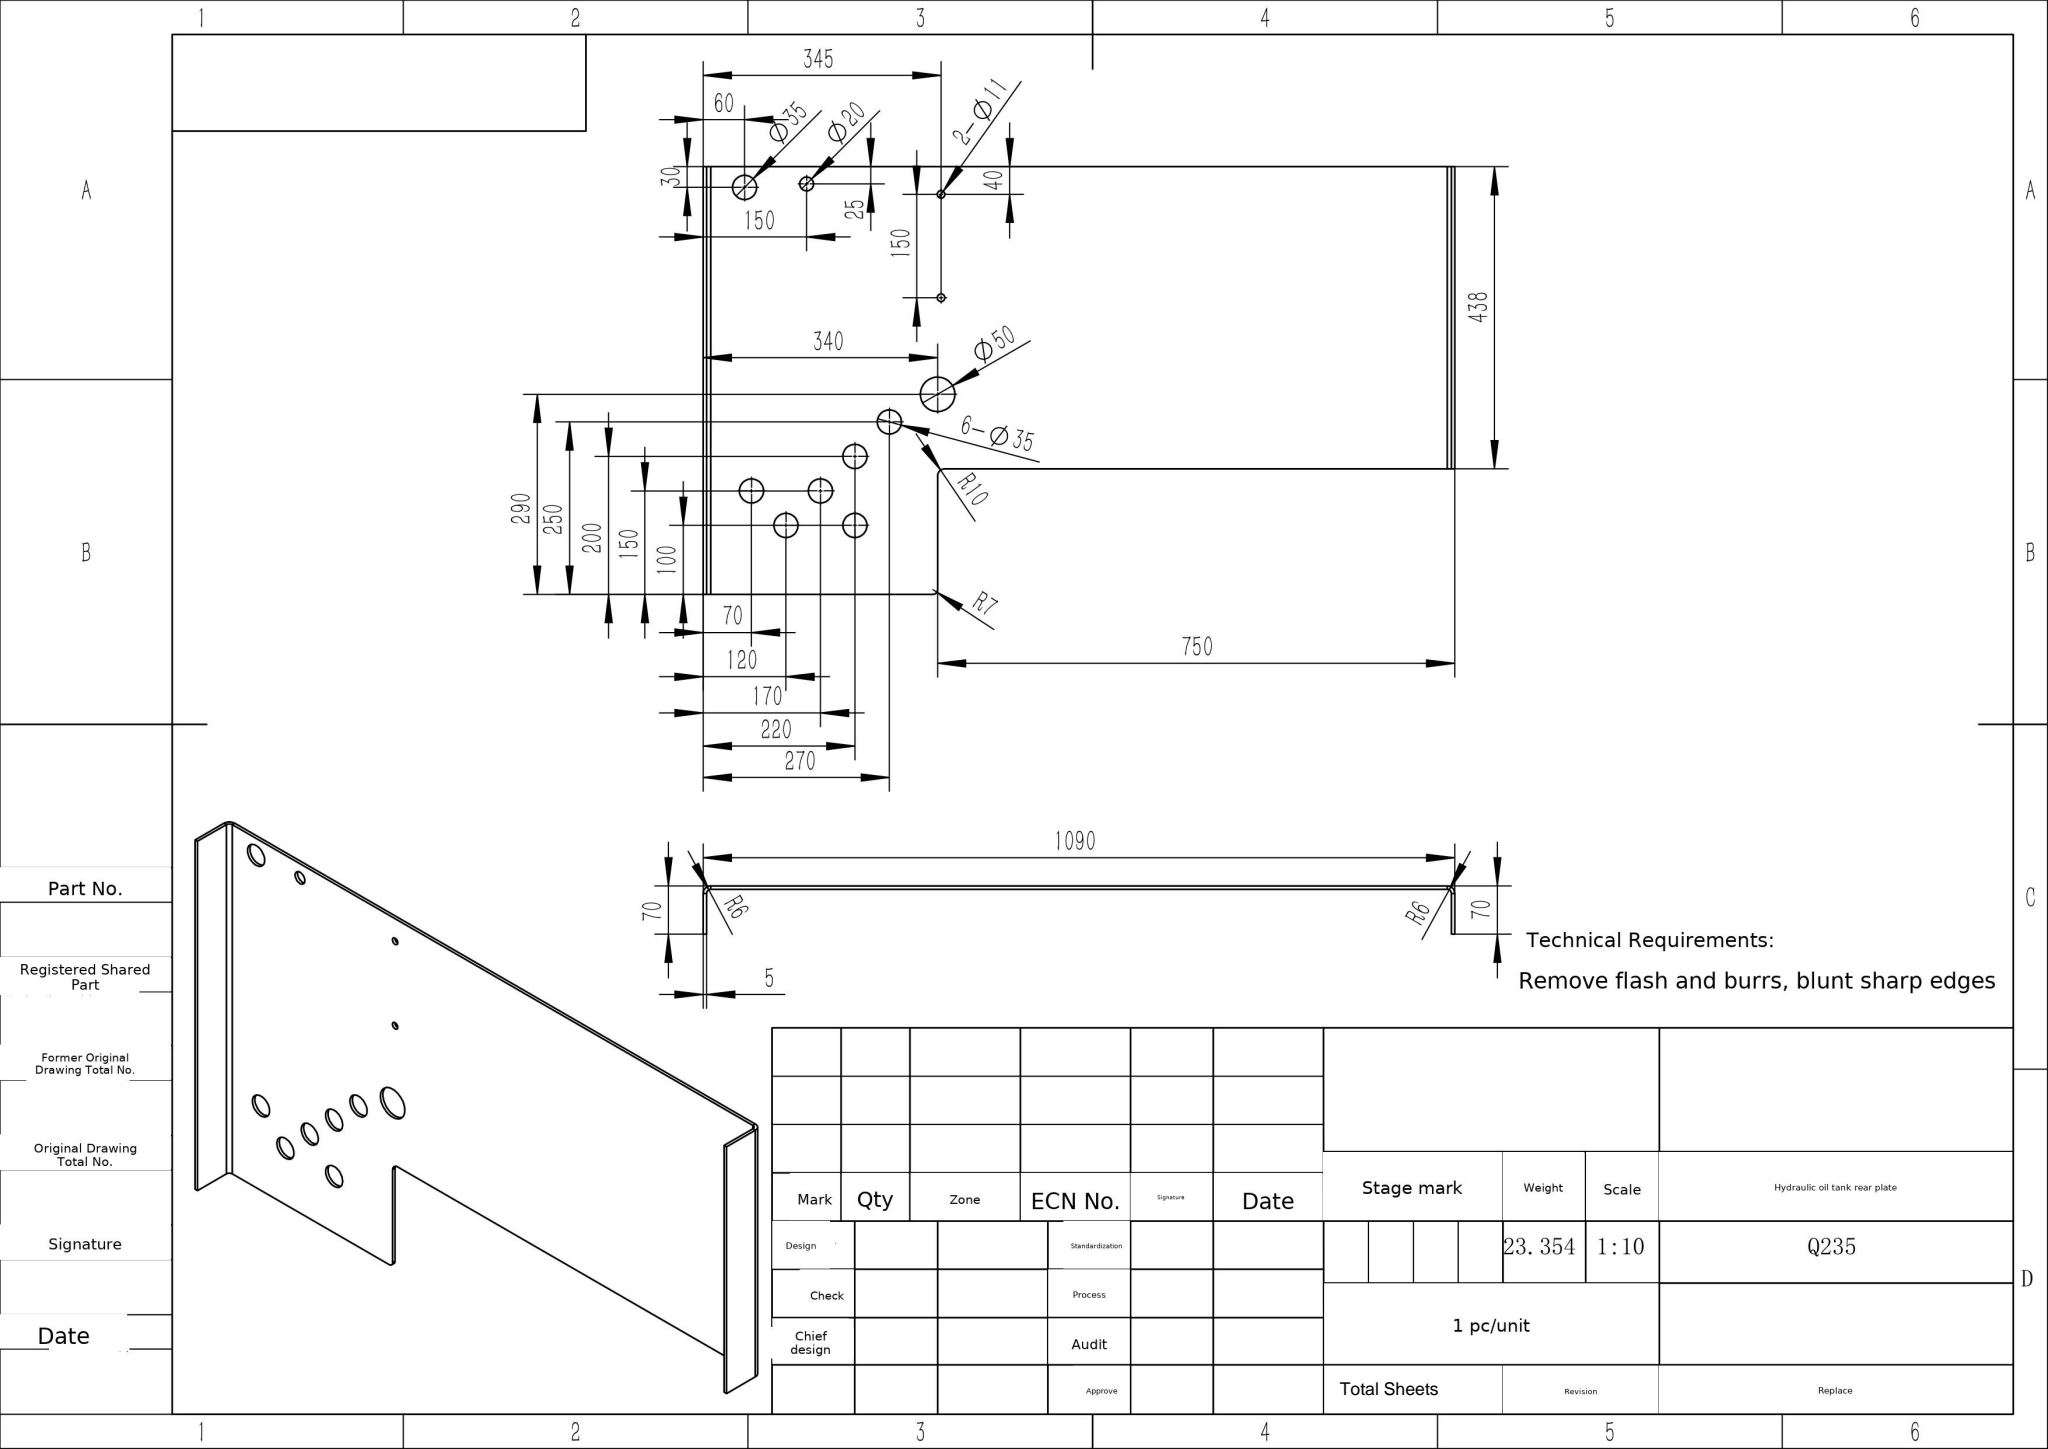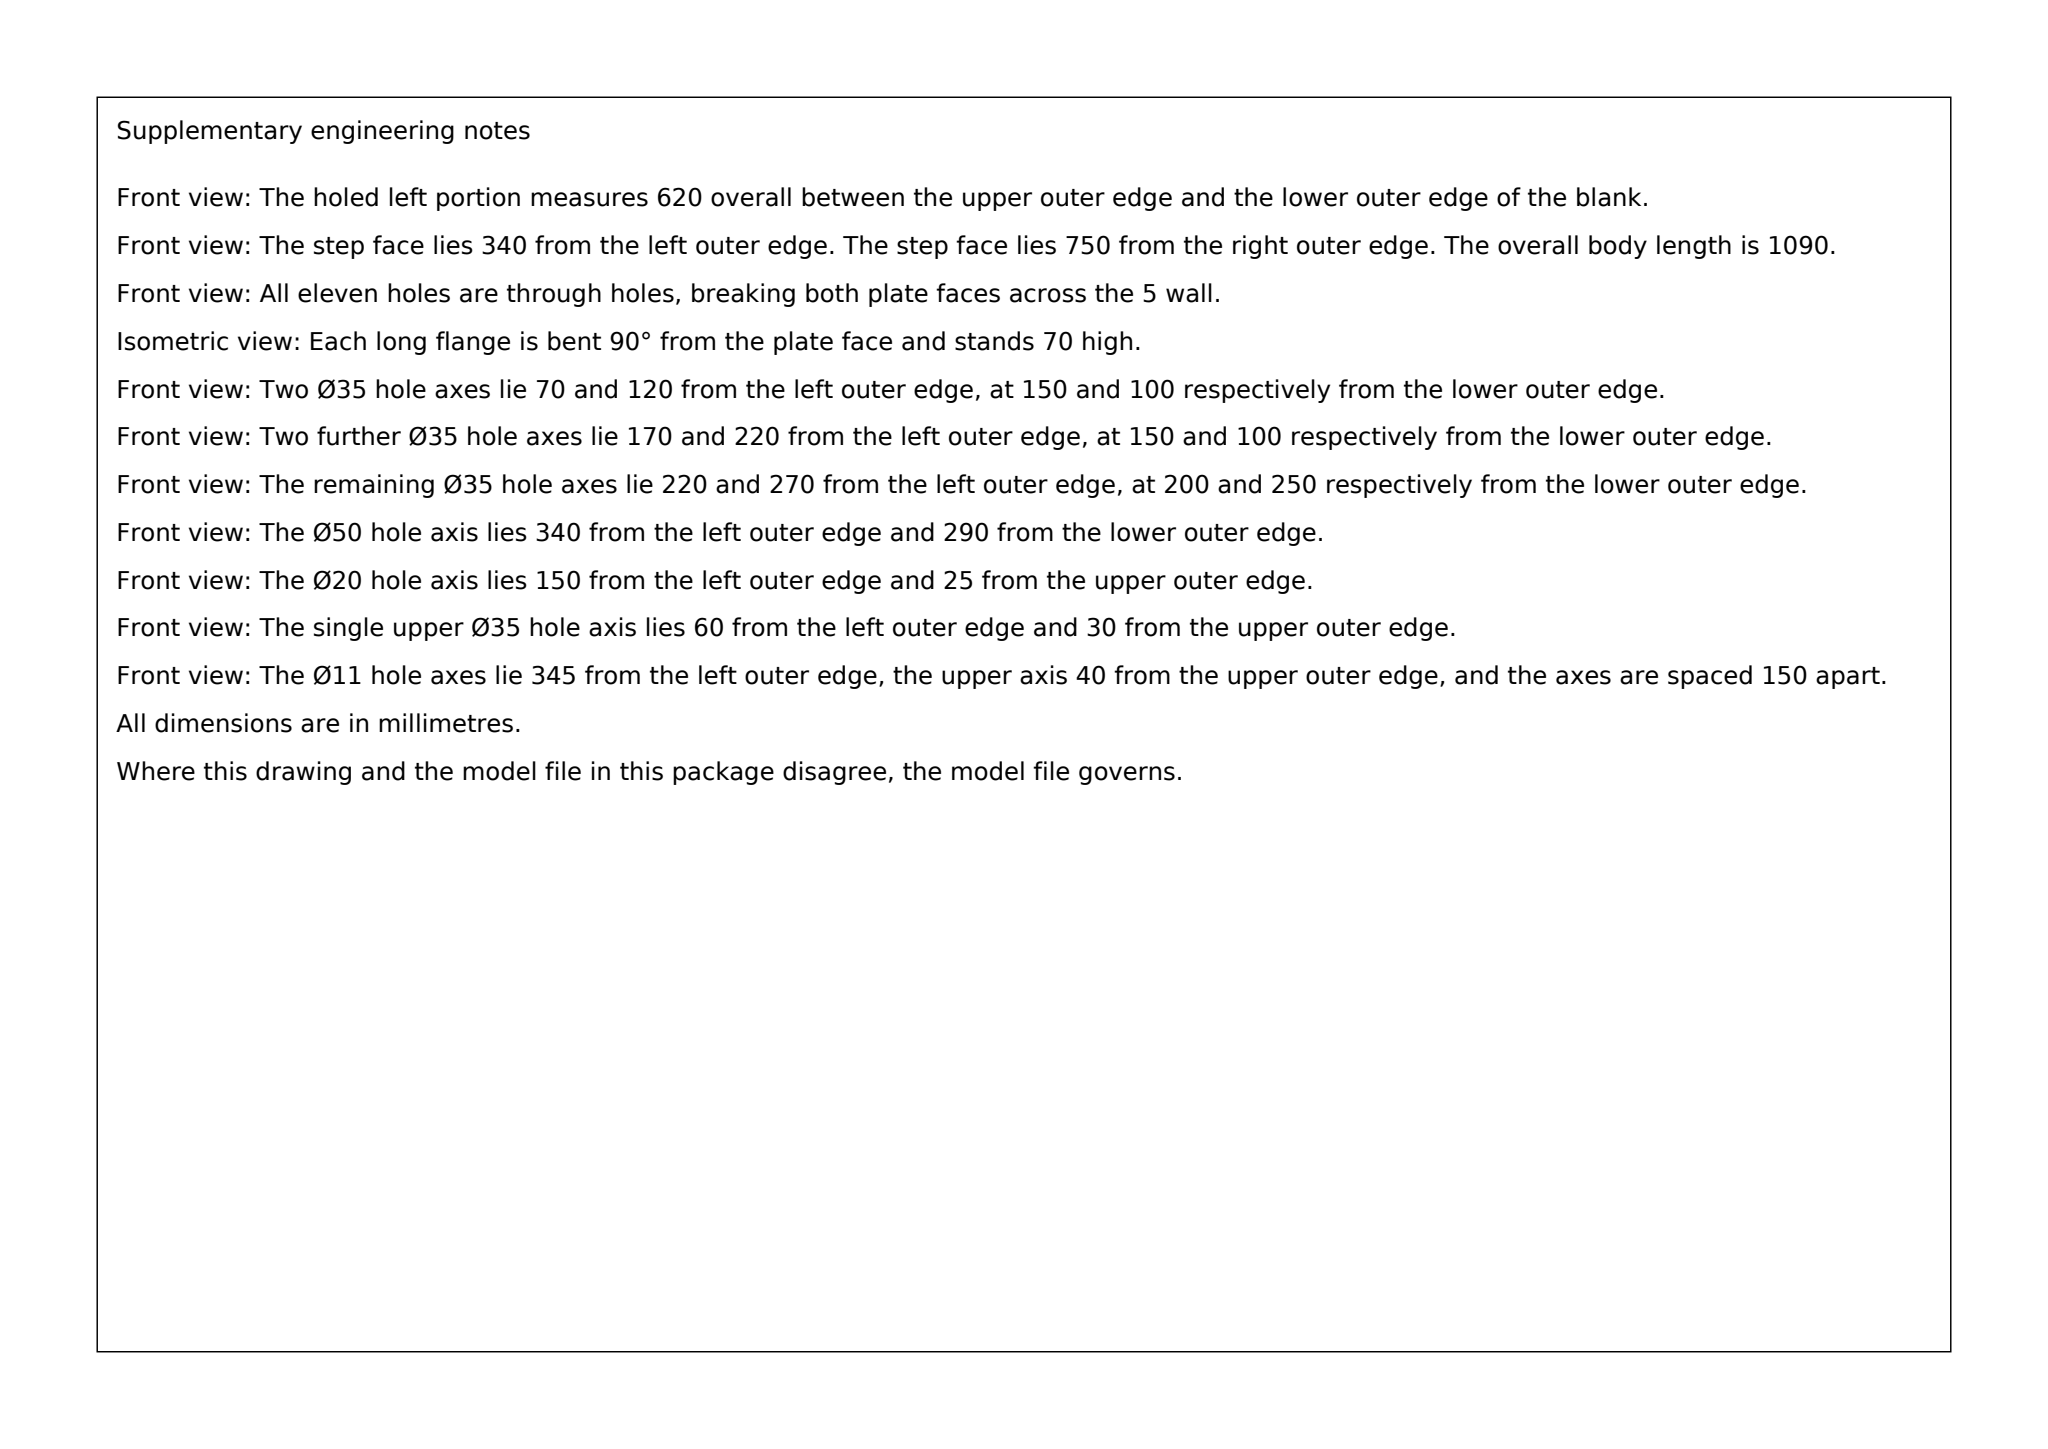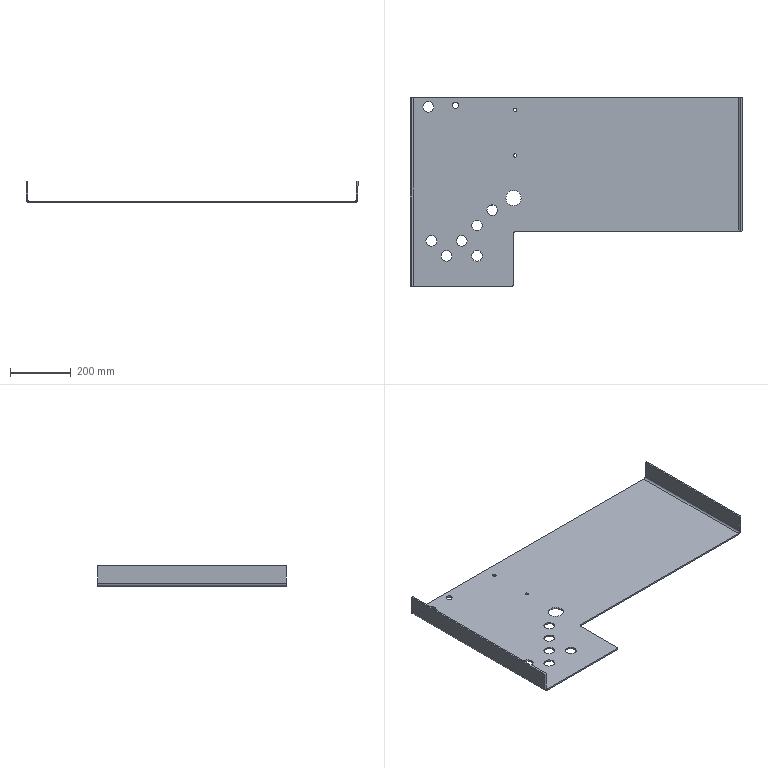Part | SolidWorks | mm | 1 solid | 48 faces | box 1090 x 620 x 70 mm | volume 2975093 mm3 | cylinder 28 | plane 20 | commonest cylinder face diameters 35 x14 11 x4 20 x3 50 x2 22 x2 12 x2 14 x1
Drawing notes:
OVERALL PLATE HT 620 (LEFT FULL-HT PORTION), FRONT VIEW | from the solid: bbox_xyz y = 620.0; planes y=0 and y=620
STEP SHOULDER 182 ABOVE BOT EDGE (= 620-438), RIGHT PORTION | from the solid: axis_plane y=182.0 with y=0 bottom and y=620 top; 620-438=182
LEFT FLANGE LG 620 FULL HT, 70 WIDE x 5 THK | from the solid: planes x=0/x=5, z=0/z=70, bbox y=620; hole dia12/22 at x=11 length 620